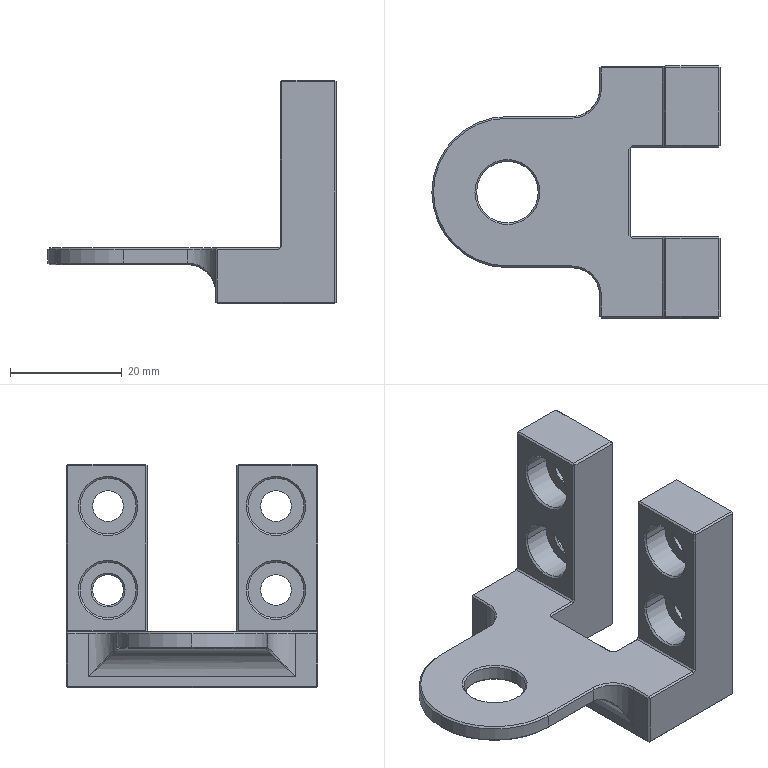Component | SolidWorks | LYB-0170-1 | 1 solid | 139 faces | volume 15835 mm3 | plane 86 | cone 28 | cylinder 23 | spline 2 | commonest cylinder face diameters 10 x11 5.5 x8 11 x2 27 x2